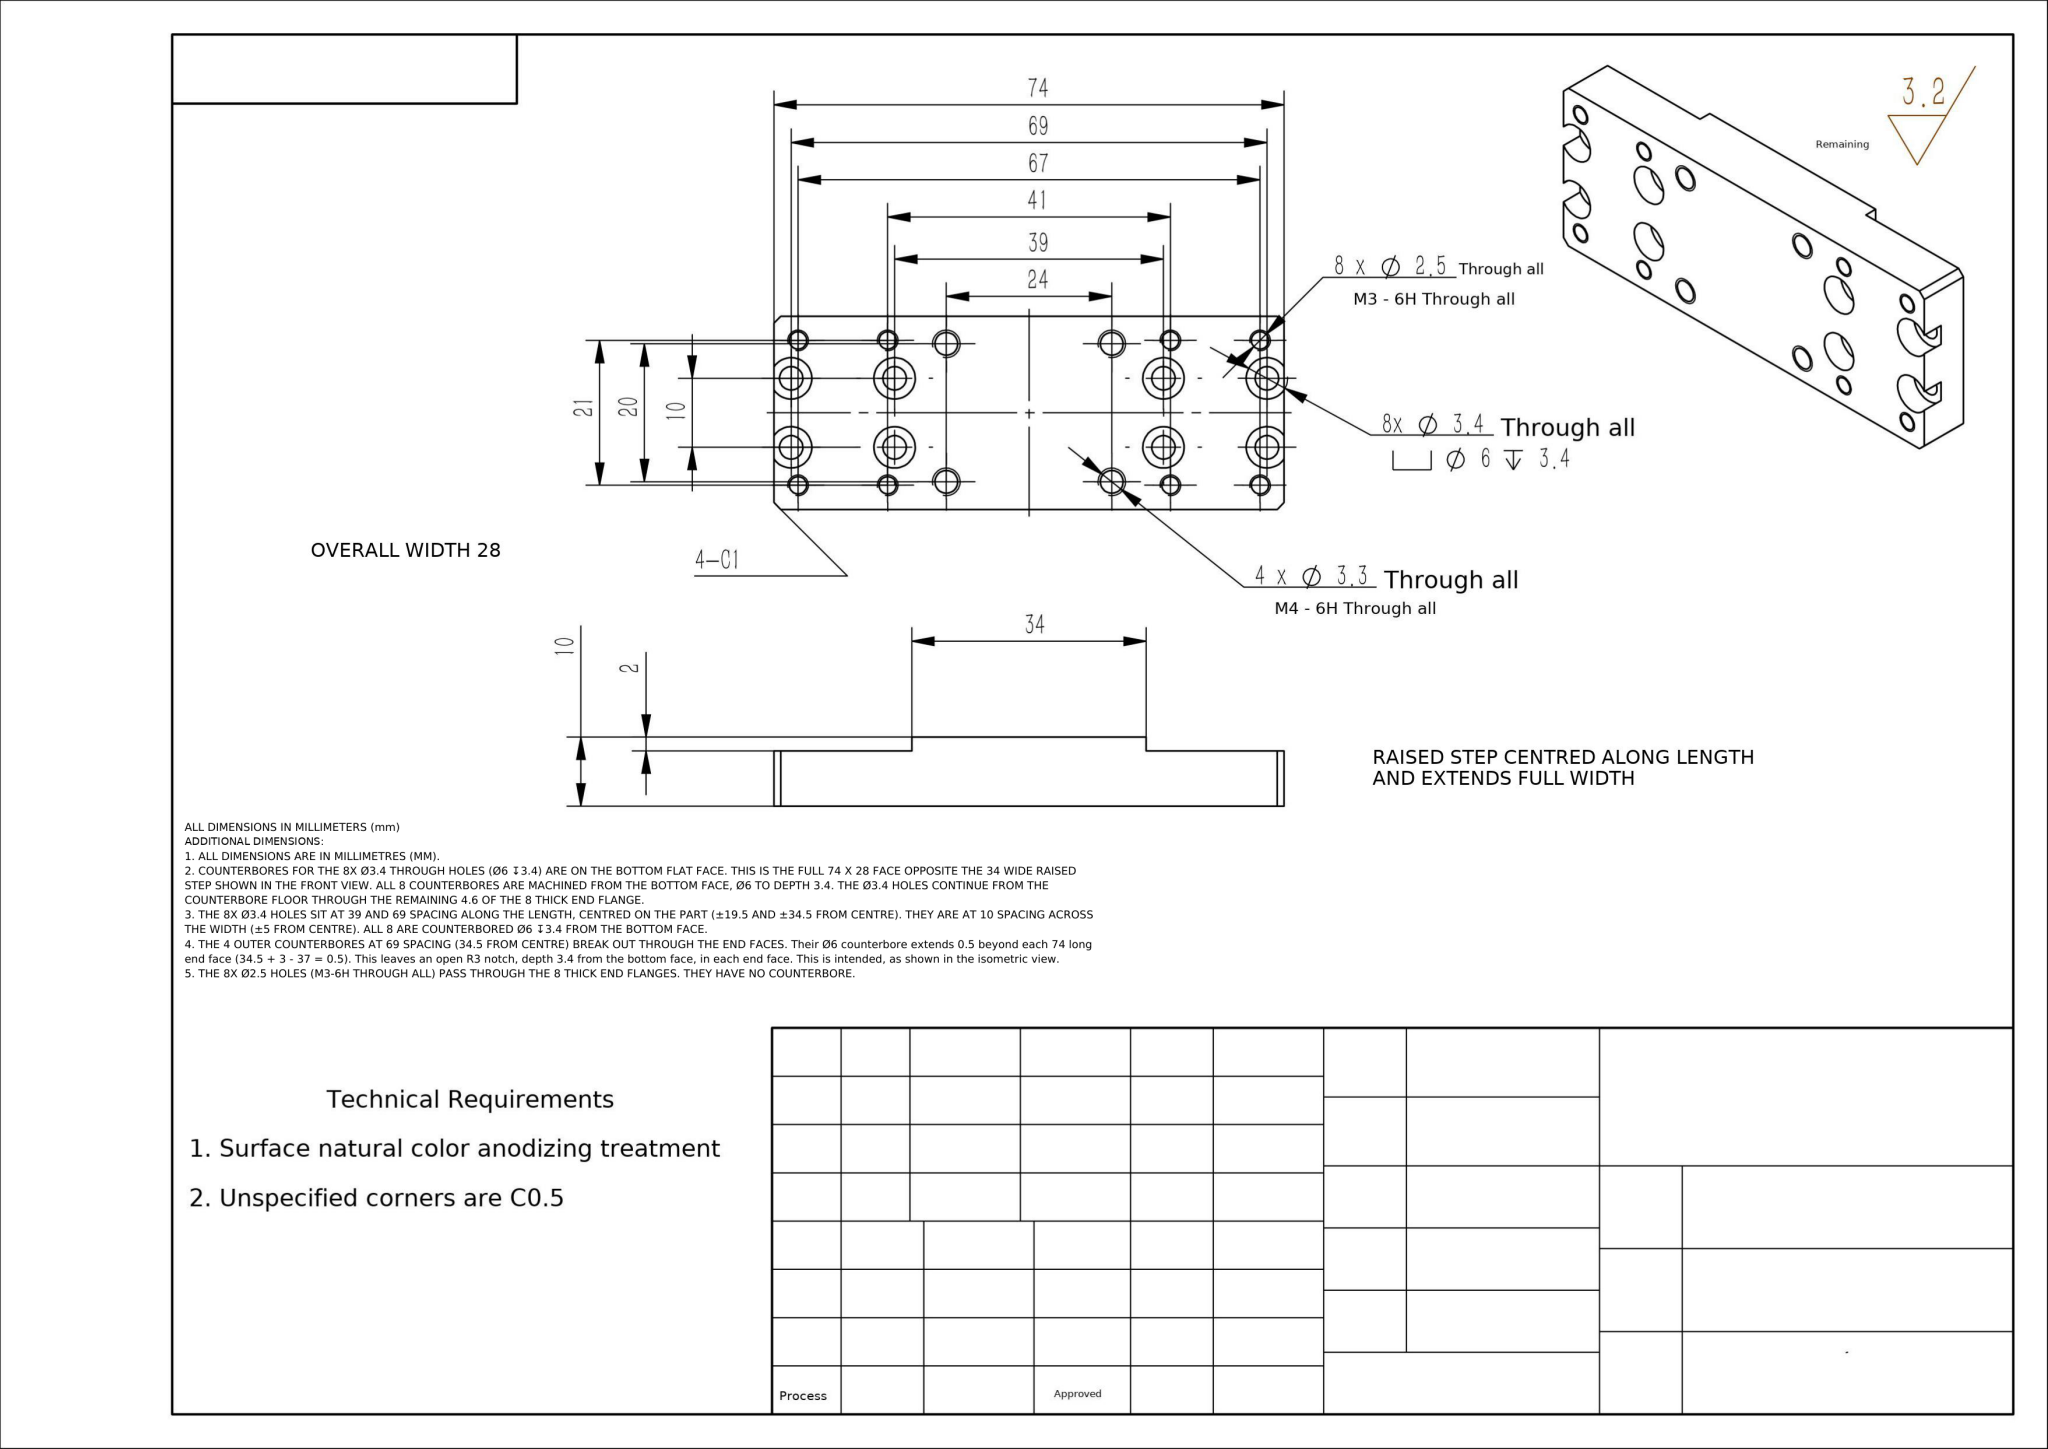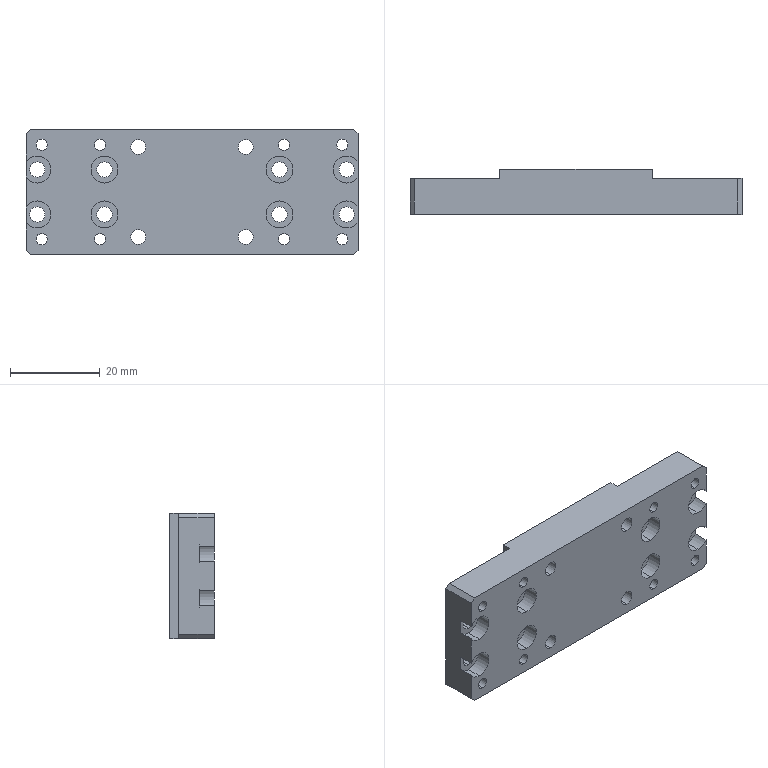Part | NX | mm | 452 | 1 solid | 82 faces | box 74 x 10 x 28 mm | volume 16720 mm3 | cylinder 60 | plane 22 | commonest cylinder face diameters 6 x20 3.4 x16 2.5 x16 3.3 x8